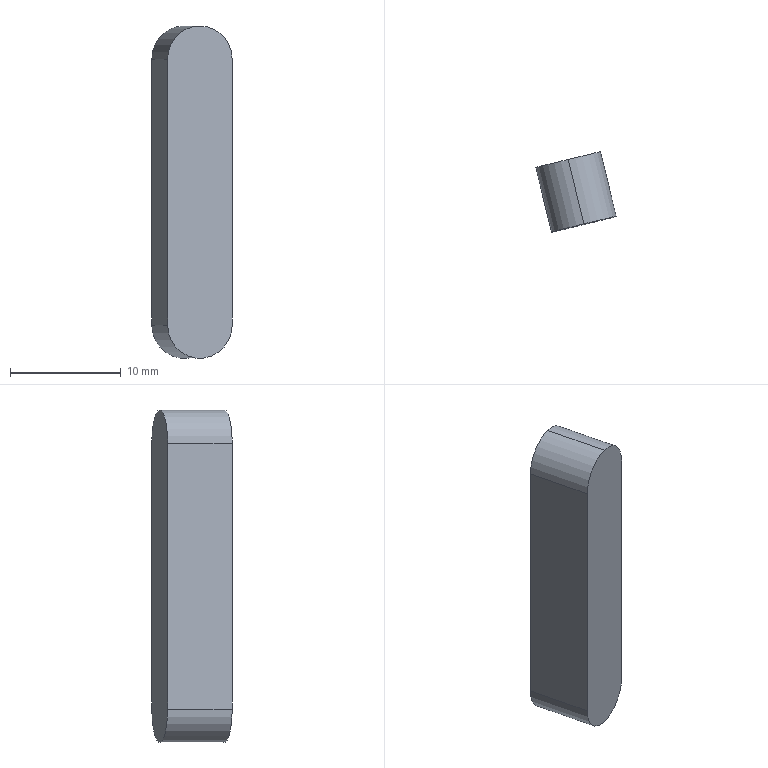Component | SolidWorks | B6-L30-1 | 1 solid | 7 faces | box 7.25 x 7.25 x 30 mm | volume 1034 mm3 | plane 4 | cylinder 3 | commonest cylinder face diameters 6 x3
build123d program:
from build123d import *

# Parameters (mm, degrees)
BOSS_EXTRUDE1_DEPTH = 6


with BuildPart() as part:
    # Sketch1 → Boss-Extrude1 (new body)
    with BuildSketch(Plane(origin=(0, 0, 0), x_dir=(-1, 0, 0), z_dir=(0, 0, -1))):
        with BuildLine():
            Line((-12, -3), (12, -3))
            ThreePointArc((12, -3), (15, 0), (12, 3))
            Line((12, 3), (-12, 3))
            ThreePointArc((-12, 3), (-15, 0), (-12, -3))
        make_face()
    extrude(amount=-BOSS_EXTRUDE1_DEPTH)


solid = part.part

# Placed as in the assembly
solid = solid.moved(Location((-20.958, -6.314, -53), (90, 13.725, -90)))
STEP:
#1=CARTESIAN_POINT('',(-0.8838,-0.5061,-1.614));
#2=VERTEX_POINT('',#1);
#3=CARTESIAN_POINT('',(-0.7691,-0.4781,-1.496));
#4=VERTEX_POINT('',#3);
#5=CARTESIAN_POINT('',(-0.7691,-0.4781,-1.614));
#6=DIRECTION('',(-0.2373,0.9714,-0.));
#7=DIRECTION('',(0.,0.,1.));
#8=AXIS2_PLACEMENT_3D('',#5,#6,#7);
#9=CIRCLE('',#8,0.1181);
#10=EDGE_CURVE('',#2,#4,#9,.T.);
#11=ORIENTED_EDGE('',*,*,#10,.T.);
#12=CARTESIAN_POINT('',(-0.8251,-0.2486,-1.496));
#13=VERTEX_POINT('',#12);
#14=CARTESIAN_POINT('',(-0.7691,-0.4781,-1.496));
#15=DIRECTION('',(-0.2373,0.9714,-0.));
#16=VECTOR('',#15,39.37);
#17=LINE('',#14,#16);
#18=EDGE_CURVE('',#4,#13,#17,.T.);
#19=ORIENTED_EDGE('',*,*,#18,.T.);
#20=CARTESIAN_POINT('',(-0.9398,-0.2766,-1.614));
#21=VERTEX_POINT('',#20);
#22=CARTESIAN_POINT('',(-0.8251,-0.2486,-1.614));
#23=DIRECTION('',(-0.2373,0.9714,-0.));
#24=DIRECTION('',(0.,0.,1.));
#25=AXIS2_PLACEMENT_3D('',#22,#23,#24);
#26=CIRCLE('',#25,0.1181);
#27=EDGE_CURVE('',#21,#13,#26,.T.);
#28=ORIENTED_EDGE('',*,*,#27,.F.);
#29=CARTESIAN_POINT('',(-0.8838,-0.5061,-1.614));
#30=DIRECTION('',(-0.2373,0.9714,-0.));
#31=VECTOR('',#30,39.37);
#32=LINE('',#29,#31);
#33=EDGE_CURVE('',#2,#21,#32,.T.);
#34=ORIENTED_EDGE('',*,*,#33,.F.);
#35=EDGE_LOOP('',(#11,#19,#28,#34));
#36=FACE_OUTER_BOUND('',#35,.T.);
#37=CARTESIAN_POINT('',(-0.7691,-0.4781,-1.614));
#38=DIRECTION('',(-0.2373,0.9714,-0.));
#39=DIRECTION('',(0.,0.,1.));
#40=AXIS2_PLACEMENT_3D('',#37,#38,#39);
#41=CYLINDRICAL_SURFACE('',#40,0.1181);
#42=ADVANCED_FACE('',(#36),#41,.T.);
#43=CARTESIAN_POINT('',(-0.7104,-0.2206,-2.559));
#44=VERTEX_POINT('',#43);
#45=CARTESIAN_POINT('',(-0.9398,-0.2766,-2.559));
#46=VERTEX_POINT('',#45);
#47=CARTESIAN_POINT('',(-0.8251,-0.2486,-2.559));
#48=DIRECTION('',(-0.2373,0.9714,-0.));
#49=DIRECTION('',(0.,0.,1.));
#50=AXIS2_PLACEMENT_3D('',#47,#48,#49);
#51=CIRCLE('',#50,0.1181);
#52=EDGE_CURVE('',#44,#46,#51,.T.);
#53=ORIENTED_EDGE('',*,*,#52,.F.);
#54=CARTESIAN_POINT('',(-0.6543,-0.4501,-2.559));
#55=VERTEX_POINT('',#54);
#56=CARTESIAN_POINT('',(-0.6543,-0.4501,-2.559));
#57=DIRECTION('',(-0.2373,0.9714,-0.));
#58=VECTOR('',#57,39.37);
#59=LINE('',#56,#58);
#60=EDGE_CURVE('',#55,#44,#59,.T.);
#61=ORIENTED_EDGE('',*,*,#60,.F.);
#62=CARTESIAN_POINT('',(-0.8838,-0.5061,-2.559));
#63=VERTEX_POINT('',#62);
#64=CARTESIAN_POINT('',(-0.7691,-0.4781,-2.559));
#65=DIRECTION('',(-0.2373,0.9714,-0.));
#66=DIRECTION('',(0.,0.,1.));
#67=AXIS2_PLACEMENT_3D('',#64,#65,#66);
#68=CIRCLE('',#67,0.1181);
#69=EDGE_CURVE('',#55,#63,#68,.T.);
#70=ORIENTED_EDGE('',*,*,#69,.T.);
#71=CARTESIAN_POINT('',(-0.8838,-0.5061,-2.559));
#72=DIRECTION('',(-0.2373,0.9714,-0.));
#73=VECTOR('',#72,39.37);
#74=LINE('',#71,#73);
#75=EDGE_CURVE('',#63,#46,#74,.T.);
#76=ORIENTED_EDGE('',*,*,#75,.T.);
#77=EDGE_LOOP('',(#53,#61,#70,#76));
#78=FACE_OUTER_BOUND('',#77,.T.);
#79=CARTESIAN_POINT('',(-0.7691,-0.4781,-2.559));
#80=DIRECTION('',(-0.2373,0.9714,-0.));
#81=DIRECTION('',(0.,0.,1.));
#82=AXIS2_PLACEMENT_3D('',#79,#80,#81);
#83=CYLINDRICAL_SURFACE('',#82,0.1181);
#84=ADVANCED_FACE('',(#78),#83,.T.);
#85=CARTESIAN_POINT('',(-0.7104,-0.2206,-1.614));
#86=VERTEX_POINT('',#85);
#87=CARTESIAN_POINT('',(-0.7104,-0.2206,-1.614));
#88=DIRECTION('',(0.,0.,-1.));
#89=VECTOR('',#88,39.37);
#90=LINE('',#87,#89);
#91=EDGE_CURVE('',#86,#44,#90,.T.);
#92=ORIENTED_EDGE('',*,*,#91,.F.);
#93=CARTESIAN_POINT('',(-0.6543,-0.4501,-1.614));
#94=VERTEX_POINT('',#93);
#95=CARTESIAN_POINT('',(-0.6543,-0.4501,-1.614));
#96=DIRECTION('',(-0.2373,0.9714,-0.));
#97=VECTOR('',#96,39.37);
#98=LINE('',#95,#97);
#99=EDGE_CURVE('',#94,#86,#98,.T.);
#100=ORIENTED_EDGE('',*,*,#99,.F.);
#101=CARTESIAN_POINT('',(-0.6543,-0.4501,-1.614));
#102=DIRECTION('',(0.,0.,-1.));
#103=VECTOR('',#102,39.37);
#104=LINE('',#101,#103);
#105=EDGE_CURVE('',#94,#55,#104,.T.);
#106=ORIENTED_EDGE('',*,*,#105,.T.);
#107=ORIENTED_EDGE('',*,*,#60,.T.);
#108=EDGE_LOOP('',(#92,#100,#106,#107));
#109=FACE_OUTER_BOUND('',#108,.T.);
#110=CARTESIAN_POINT('',(-0.6543,-0.4501,-1.614));
#111=DIRECTION('',(0.9714,0.2373,0.));
#112=DIRECTION('',(0.2373,-0.9714,0.));
#113=AXIS2_PLACEMENT_3D('',#110,#111,#112);
#114=PLANE('',#113);
#115=ADVANCED_FACE('',(#109),#114,.T.);
#116=ORIENTED_EDGE('',*,*,#18,.F.);
#117=CARTESIAN_POINT('',(-0.7691,-0.4781,-1.614));
#118=DIRECTION('',(-0.2373,0.9714,-0.));
#119=DIRECTION('',(0.,0.,1.));
#120=AXIS2_PLACEMENT_3D('',#117,#118,#119);
#121=CIRCLE('',#120,0.1181);
#122=EDGE_CURVE('',#4,#94,#121,.T.);
#123=ORIENTED_EDGE('',*,*,#122,.T.);
#124=ORIENTED_EDGE('',*,*,#99,.T.);
#125=CARTESIAN_POINT('',(-0.8251,-0.2486,-1.614));
#126=DIRECTION('',(-0.2373,0.9714,-0.));
#127=DIRECTION('',(0.,0.,1.));
#128=AXIS2_PLACEMENT_3D('',#125,#126,#127);
#129=CIRCLE('',#128,0.1181);
#130=EDGE_CURVE('',#13,#86,#129,.T.);
#131=ORIENTED_EDGE('',*,*,#130,.F.);
#132=EDGE_LOOP('',(#116,#123,#124,#131));
#133=FACE_OUTER_BOUND('',#132,.T.);
#134=CARTESIAN_POINT('',(-0.7691,-0.4781,-1.614));
#135=DIRECTION('',(-0.2373,0.9714,-0.));
#136=DIRECTION('',(0.,0.,1.));
#137=AXIS2_PLACEMENT_3D('',#134,#135,#136);
#138=CYLINDRICAL_SURFACE('',#137,0.1181);
#139=ADVANCED_FACE('',(#133),#138,.T.);
#140=CARTESIAN_POINT('',(-0.9398,-0.2766,-2.559));
#141=DIRECTION('',(-0.,-0.,1.));
#142=VECTOR('',#141,39.37);
#143=LINE('',#140,#142);
#144=EDGE_CURVE('',#46,#21,#143,.T.);
#145=ORIENTED_EDGE('',*,*,#144,.F.);
#146=ORIENTED_EDGE('',*,*,#75,.F.);
#147=CARTESIAN_POINT('',(-0.8838,-0.5061,-2.559));
#148=DIRECTION('',(-0.,-0.,1.));
#149=VECTOR('',#148,39.37);
#150=LINE('',#147,#149);
#151=EDGE_CURVE('',#63,#2,#150,.T.);
#152=ORIENTED_EDGE('',*,*,#151,.T.);
#153=ORIENTED_EDGE('',*,*,#33,.T.);
#154=EDGE_LOOP('',(#145,#146,#152,#153));
#155=FACE_OUTER_BOUND('',#154,.T.);
#156=CARTESIAN_POINT('',(-0.8838,-0.5061,-2.559));
#157=DIRECTION('',(-0.9714,-0.2373,-0.));
#158=DIRECTION('',(-0.2373,0.9714,-0.));
#159=AXIS2_PLACEMENT_3D('',#156,#157,#158);
#160=PLANE('',#159);
#161=ADVANCED_FACE('',(#155),#160,.T.);
#162=ORIENTED_EDGE('',*,*,#69,.F.);
#163=ORIENTED_EDGE('',*,*,#105,.F.);
#164=ORIENTED_EDGE('',*,*,#122,.F.);
#165=ORIENTED_EDGE('',*,*,#10,.F.);
#166=ORIENTED_EDGE('',*,*,#151,.F.);
#167=EDGE_LOOP('',(#162,#163,#164,#165,#166));
#168=FACE_OUTER_BOUND('',#167,.T.);
#169=CARTESIAN_POINT('',(-0.7691,-0.4781,-2.559));
#170=DIRECTION('',(-0.2373,0.9714,-0.));
#171=DIRECTION('',(-0.,-0.,1.));
#172=AXIS2_PLACEMENT_3D('',#169,#170,#171);
#173=PLANE('',#172);
#174=ADVANCED_FACE('',(#168),#173,.F.);
#175=ORIENTED_EDGE('',*,*,#52,.T.);
#176=ORIENTED_EDGE('',*,*,#144,.T.);
#177=ORIENTED_EDGE('',*,*,#27,.T.);
#178=ORIENTED_EDGE('',*,*,#130,.T.);
#179=ORIENTED_EDGE('',*,*,#91,.T.);
#180=EDGE_LOOP('',(#175,#176,#177,#178,#179));
#181=FACE_OUTER_BOUND('',#180,.T.);
#182=CARTESIAN_POINT('',(-0.8251,-0.2486,-2.559));
#183=DIRECTION('',(-0.2373,0.9714,-0.));
#184=DIRECTION('',(-0.,-0.,1.));
#185=AXIS2_PLACEMENT_3D('',#182,#183,#184);
#186=PLANE('',#185);
#187=ADVANCED_FACE('',(#181),#186,.T.);
#188=CLOSED_SHELL('',(#42,#84,#115,#139,#161,#174,#187));
#189=MANIFOLD_SOLID_BREP('',#188);
#190=CARTESIAN_POINT('',(0.,0.,0.));
#191=DIRECTION('',(0.,0.,1.));
#192=DIRECTION('',(1.,0.,0.));
#193=AXIS2_PLACEMENT_3D('',#190,#191,#192);
#194=(LENGTH_UNIT()NAMED_UNIT(*)SI_UNIT($,.METRE.));
#195=LENGTH_MEASURE_WITH_UNIT(LENGTH_MEASURE(0.0254),#194);
#196=DIMENSIONAL_EXPONENTS(1.,0.,0.,0.,0.,0.,0.);
#197=(CONVERSION_BASED_UNIT('',#195)LENGTH_UNIT()NAMED_UNIT(#196));
#198=UNCERTAINTY_MEASURE_WITH_UNIT(LENGTH_MEASURE(0.00001),#197,'','');
#199=(NAMED_UNIT(*)PLANE_ANGLE_UNIT()SI_UNIT($,.RADIAN.));
#200=(NAMED_UNIT(*)SI_UNIT($,.STERADIAN.)SOLID_ANGLE_UNIT());
#201=(GEOMETRIC_REPRESENTATION_CONTEXT(3)GLOBAL_UNCERTAINTY_ASSIGNED_CONTEXT((#198))GLOBAL_UNIT_ASSIGNED_CONTEXT((#197,#199,#200))REPRESENTATION_CONTEXT('',''));
#202=ADVANCED_BREP_SHAPE_REPRESENTATION('',(#189,#193),#201);
#203=COLOUR_RGB('',0.7922,0.8196,0.9333);
#204=FILL_AREA_STYLE_COLOUR('',#203);
#205=FILL_AREA_STYLE('',(#204));
#206=SURFACE_STYLE_FILL_AREA(#205);
#207=SURFACE_SIDE_STYLE('',(#206));
#208=SURFACE_STYLE_USAGE(.BOTH.,#207);
#209=PRESENTATION_STYLE_ASSIGNMENT((#208));
#210=STYLED_ITEM('',(#209),#189);
#211=PRESENTATION_LAYER_ASSIGNMENT('','',(#210));
#212=(LENGTH_UNIT()NAMED_UNIT(*)SI_UNIT($,.METRE.));
#213=LENGTH_MEASURE_WITH_UNIT(LENGTH_MEASURE(0.0254),#212);
#214=DIMENSIONAL_EXPONENTS(1.,0.,0.,0.,0.,0.,0.);
#215=(CONVERSION_BASED_UNIT('',#213)LENGTH_UNIT()NAMED_UNIT(#214));
#216=UNCERTAINTY_MEASURE_WITH_UNIT(LENGTH_MEASURE(0.00001),#215,'','');
#217=(NAMED_UNIT(*)PLANE_ANGLE_UNIT()SI_UNIT($,.RADIAN.));
#218=(NAMED_UNIT(*)SI_UNIT($,.STERADIAN.)SOLID_ANGLE_UNIT());
#219=(GEOMETRIC_REPRESENTATION_CONTEXT(3)GLOBAL_UNCERTAINTY_ASSIGNED_CONTEXT((#216))GLOBAL_UNIT_ASSIGNED_CONTEXT((#215,#217,#218))REPRESENTATION_CONTEXT('',''));
#220=MECHANICAL_DESIGN_GEOMETRIC_PRESENTATION_REPRESENTATION('',(#210),#219);